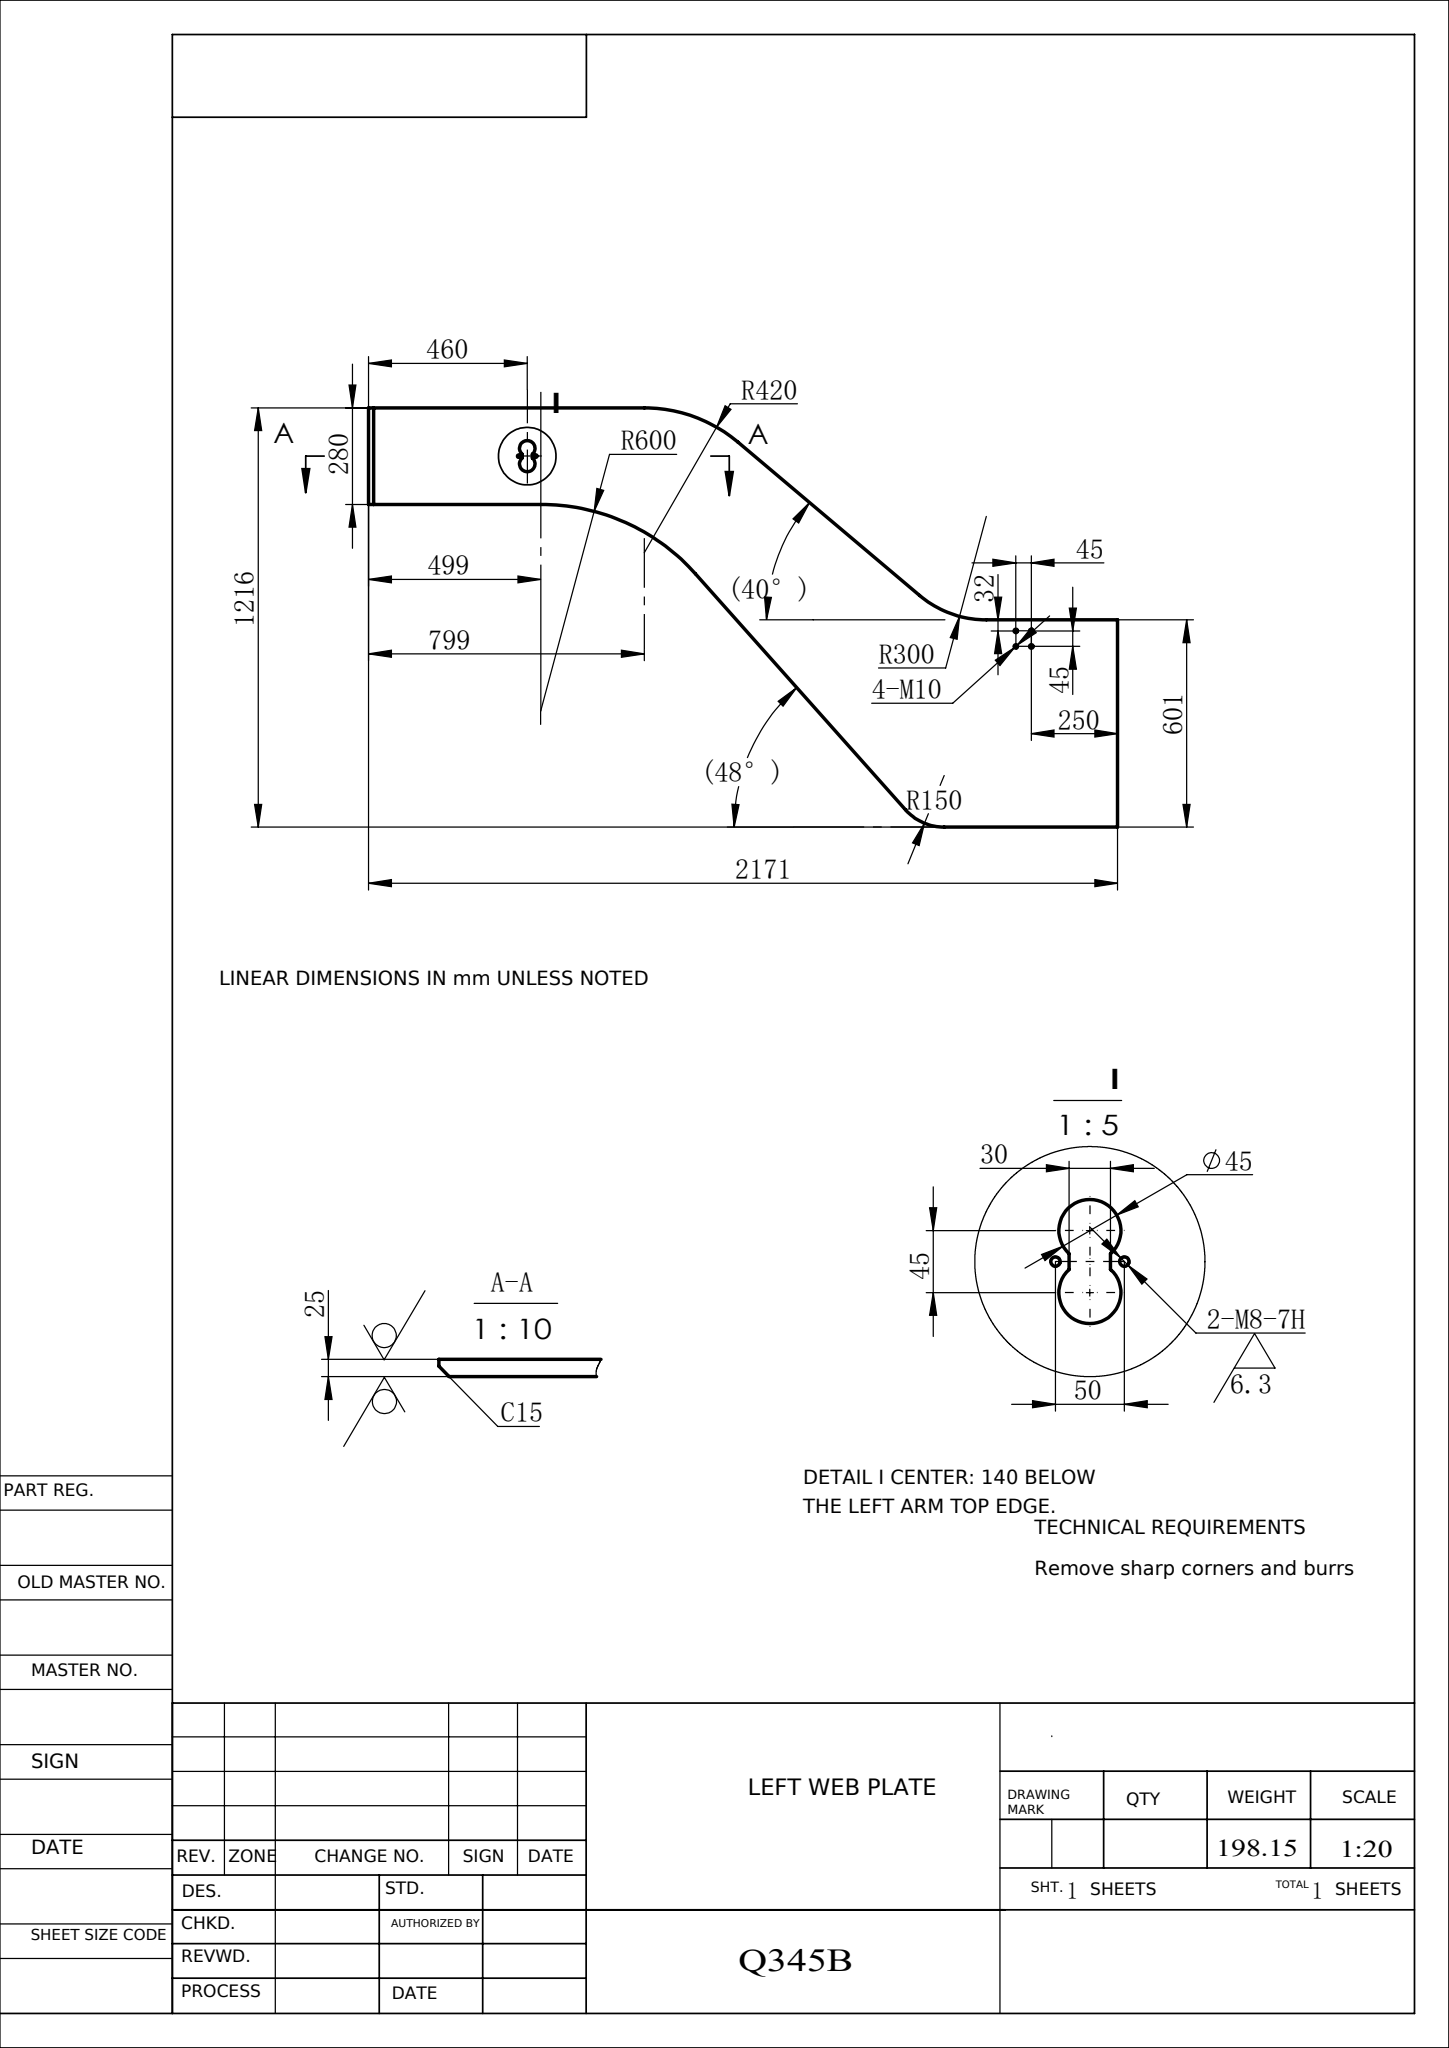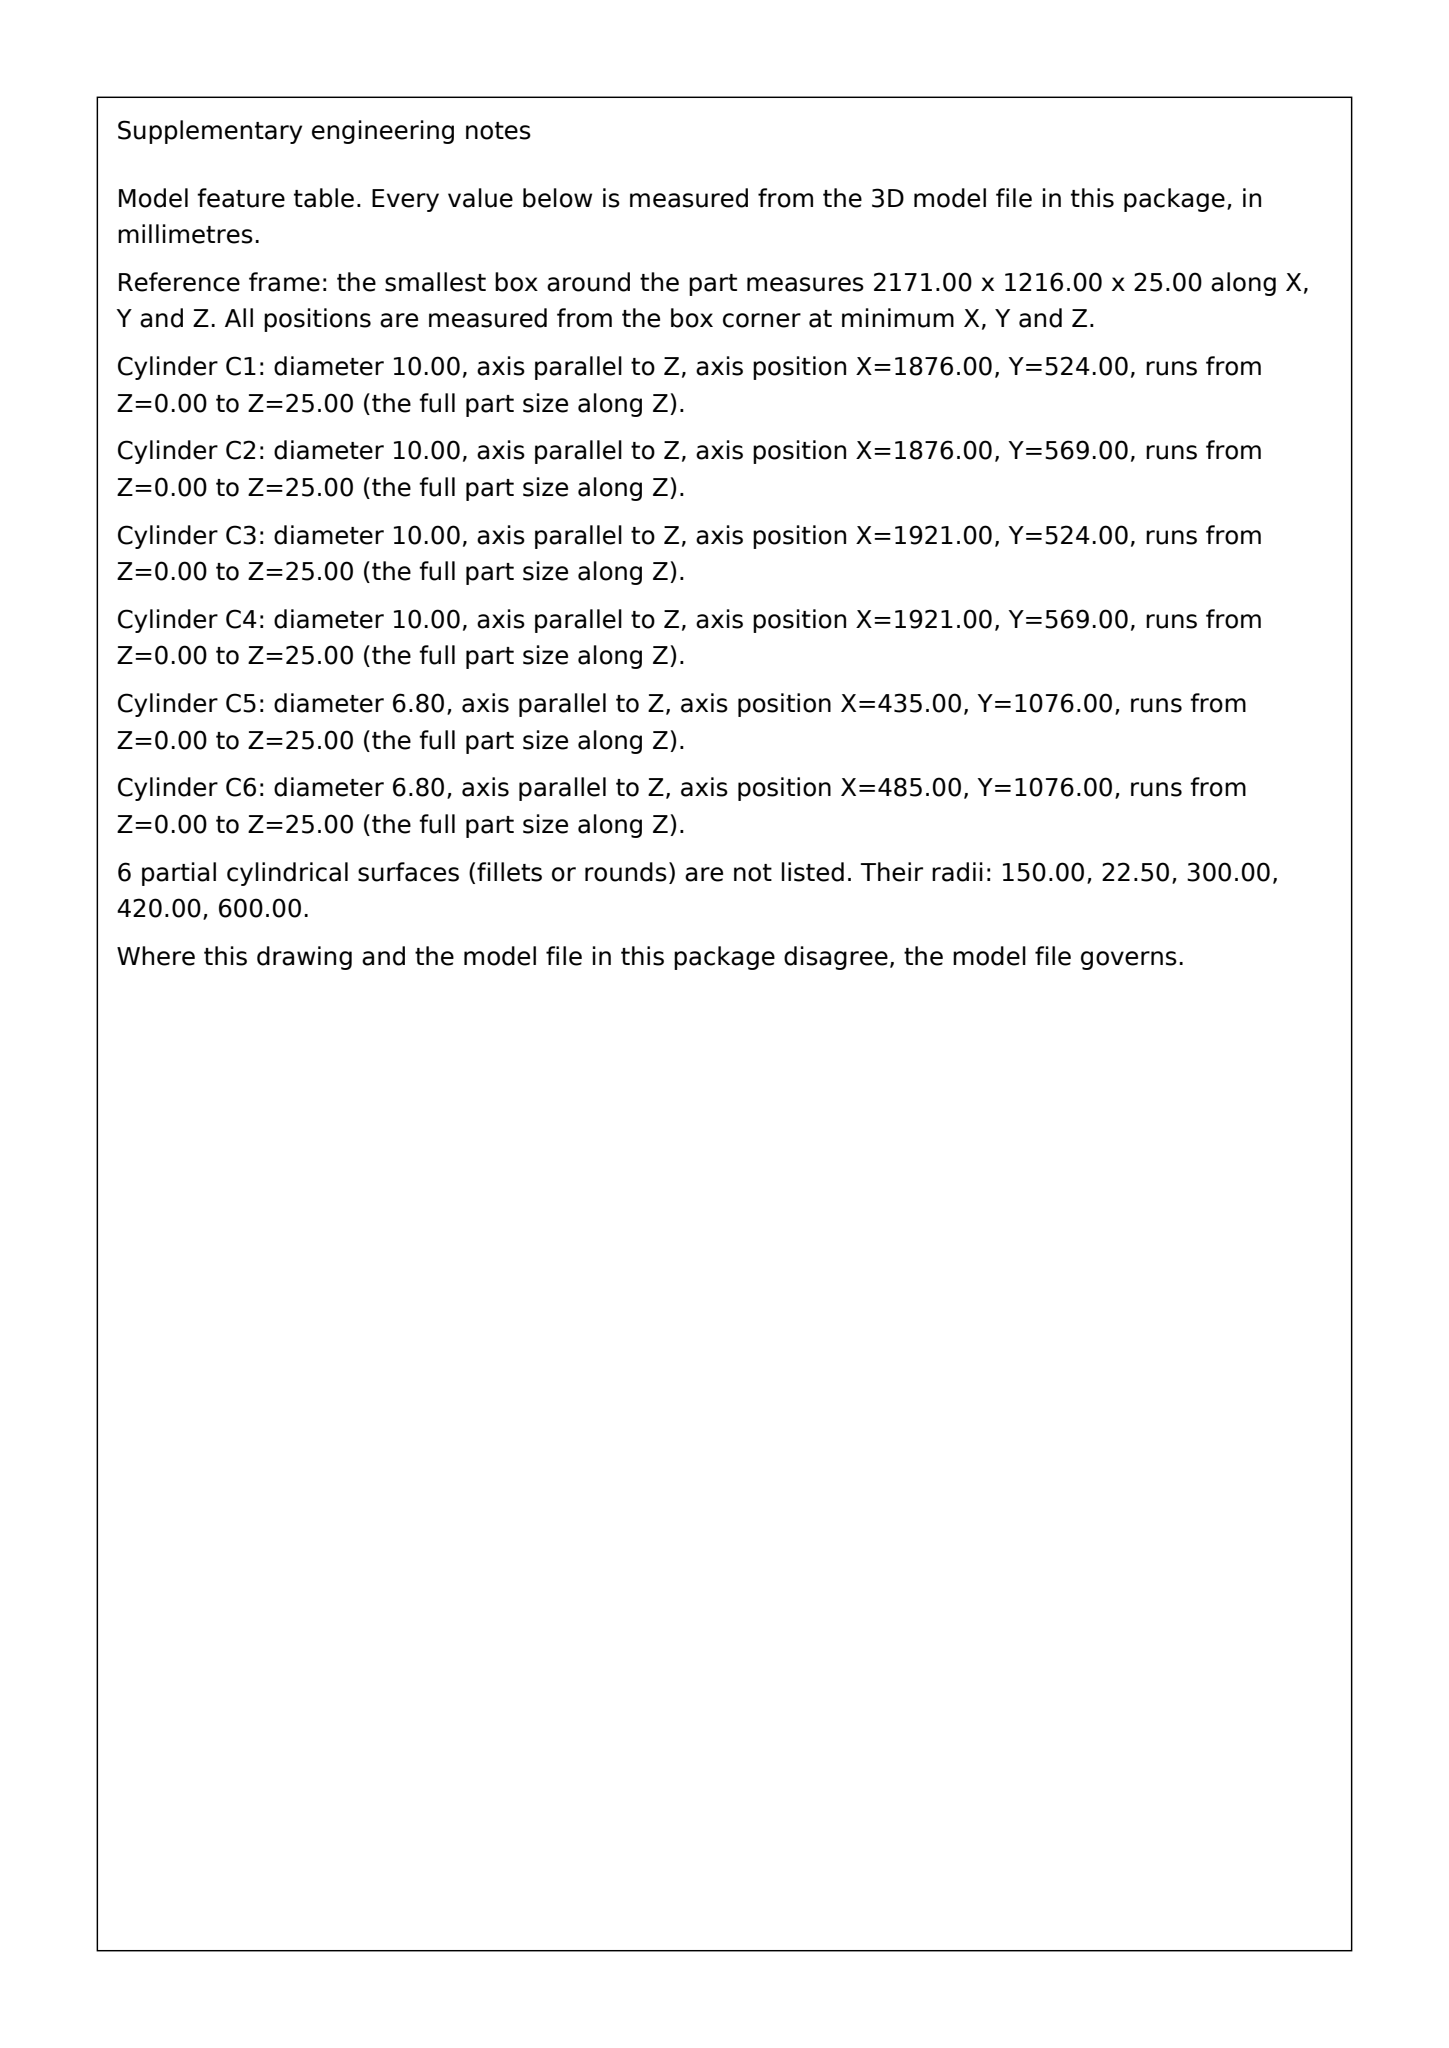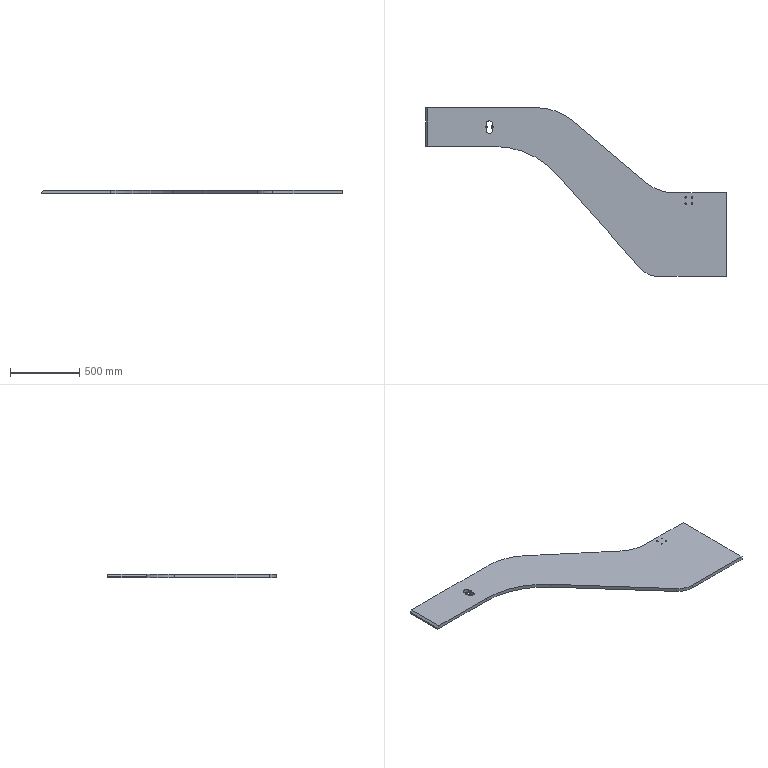Part | SolidWorks | mm | material Q345B | 1 solid | 35 faces | box 2171 x 1216 x 25 mm | volume 25215707 mm3 | cylinder 22 | plane 13 | commonest cylinder face diameters 10 x8 45 x6 6.8 x4 1200 x1 840 x1 600 x1 300 x1
build123d program:
from build123d import *

# Parameters (mm, degrees)
BOSS_EXTRUDE1_DEPTH = 25
CHAMFER1_SIZE       = 15
CUT_EXTRUDE1_DEPTH  = 2365.31
FILLET1_R           = 300
FILLET2_R           = 150
M8_TAPPED_HOLE1_D   = 6.8
SKETCH5_R           = 5
CUT_EXTRUDE2_DEPTH  = 2365.31


with BuildPart() as part:
    # Sketch1 → Boss-Extrude1 (new body)
    with BuildSketch(Plane.XY):
        with BuildLine():
            Line((0, 0), (0, 280))
            Line((0, 280), (799, 280))
            ThreePointArc((799, 280), (943.25, 254.451), (1069.95, 180.914))
            Line((1069.95, 180.914), (1681, -335))
            Line((1681, -335), (2171, -335))
            Line((2171, -335), (2171, -936))
            Line((2171, -936), (1601, -936))
            Line((1601, -936), (947.276, -201.191))
            ThreePointArc((947.276, -201.191), (744.677, -52.604), (499, 0))
            Line((499, 0), (0, 0))
        make_face()
    extrude(amount=BOSS_EXTRUDE1_DEPTH)

    # Chamfer1
    chamfer1_edges = [part.edges().sort_by_distance(p)[0] for p in [
        (0, 140, 25),
    ]]
    chamfer(chamfer1_edges, length=CHAMFER1_SIZE)

    # Sketch2 → Cut-Extrude1 (cut, through all)
    with BuildSketch(Plane.XY.offset(25)):
        with BuildLine():
            Line((445, 145.729), (445, 134.271))
            ThreePointArc((445, 134.271), (460, 95), (475, 134.271))
            Line((475, 134.271), (475, 145.729))
            ThreePointArc((475, 145.729), (460, 185), (445, 145.729))
        make_face()
    extrude(amount=-CUT_EXTRUDE1_DEPTH, mode=Mode.SUBTRACT)

    # Fillet1
    fillet1_edges = [part.edges().sort_by_distance(p)[0] for p in [
        (1681, -335, 12.5),
    ]]
    fillet(fillet1_edges, radius=FILLET1_R)

    # Fillet2
    fillet2_edges = [part.edges().sort_by_distance(p)[0] for p in [
        (1601, -936, 12.5),
    ]]
    fillet(fillet2_edges, radius=FILLET2_R)

    # M8 Tapped Hole1 (through all)
    with Locations(Plane.XY.offset(25)):
        with Locations((435, 140), (485, 140)):
            Hole(M8_TAPPED_HOLE1_D / 2)

    # Sketch5 → Cut-Extrude2 (cut, through all)
    with BuildSketch(Plane.XY.offset(25)):
        with Locations((1876, -367)):
            Circle(SKETCH5_R)
        with Locations((1921, -367)):
            Circle(SKETCH5_R)
        with Locations((1876, -412)):
            Circle(SKETCH5_R)
        with Locations((1921, -412)):
            Circle(SKETCH5_R)
    extrude(amount=-CUT_EXTRUDE2_DEPTH, mode=Mode.SUBTRACT)


solid = part.part